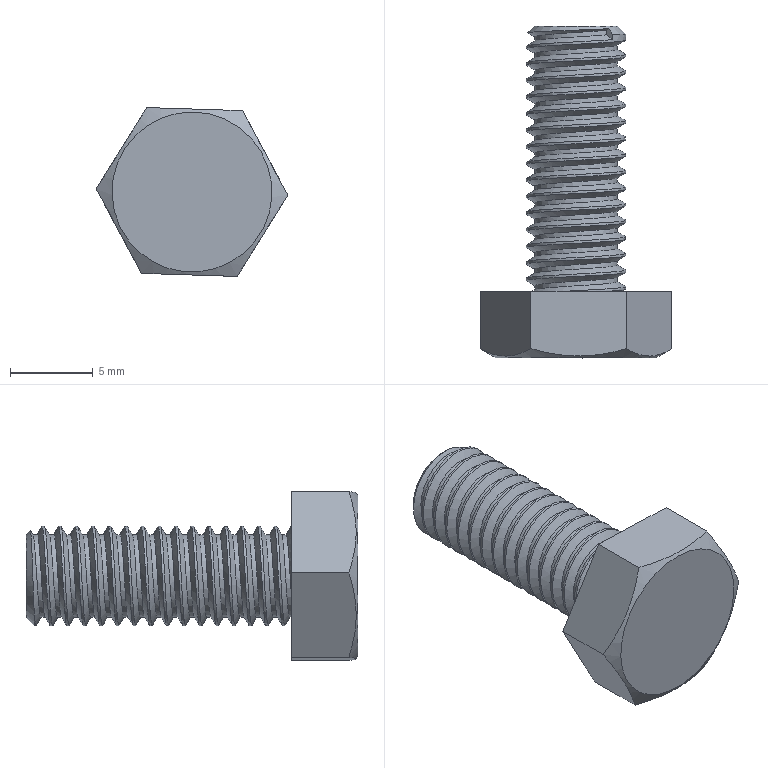Component | NX | BOLT_2 | 1 solid | 16 faces | volume 718 mm3 | plane 10 | cylinder 2 | spline 2 | cone 2 | commonest cylinder face diameters 6 x1 5 x1